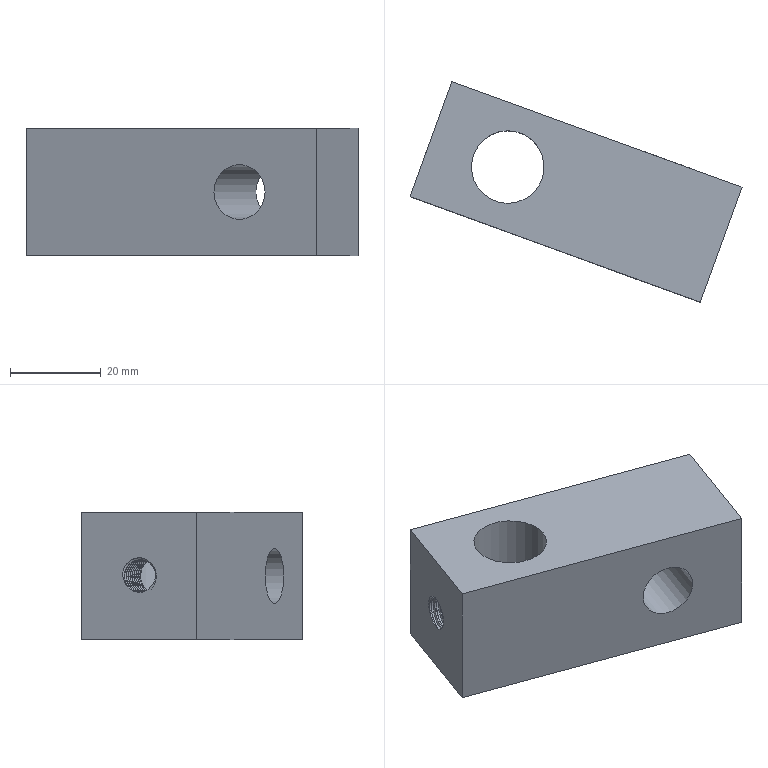Component | NX | 4 | 1 solid | 15 faces | volume 42258 mm3 | plane 7 | cylinder 5 | spline 3 | commonest cylinder face diameters 7.188 x2 16 x1 12 x1 8 x1